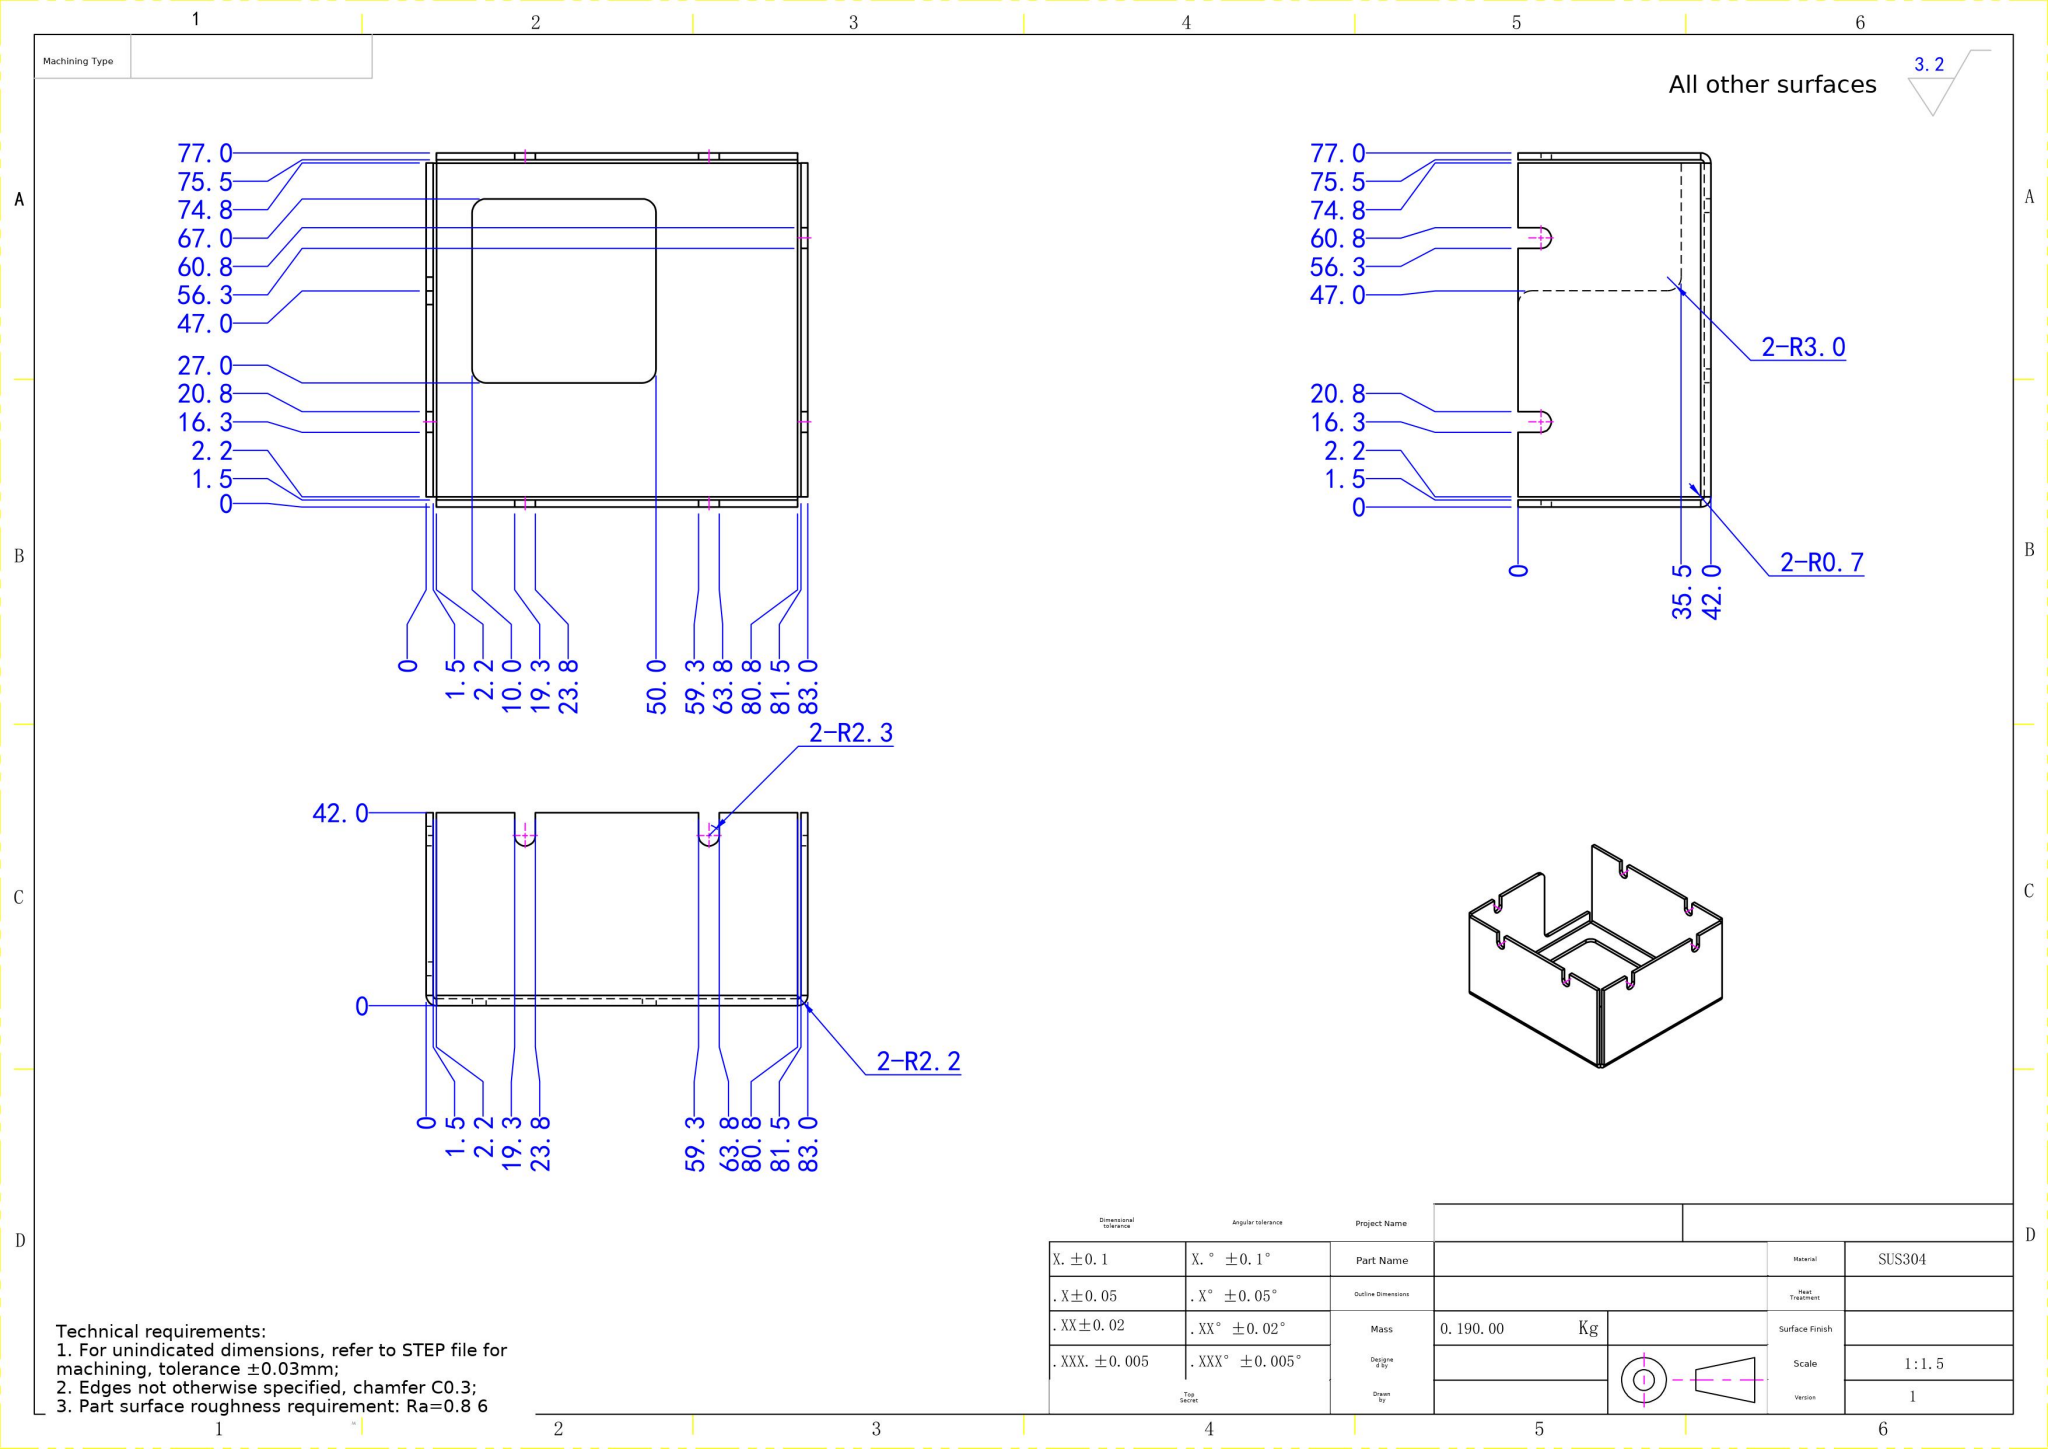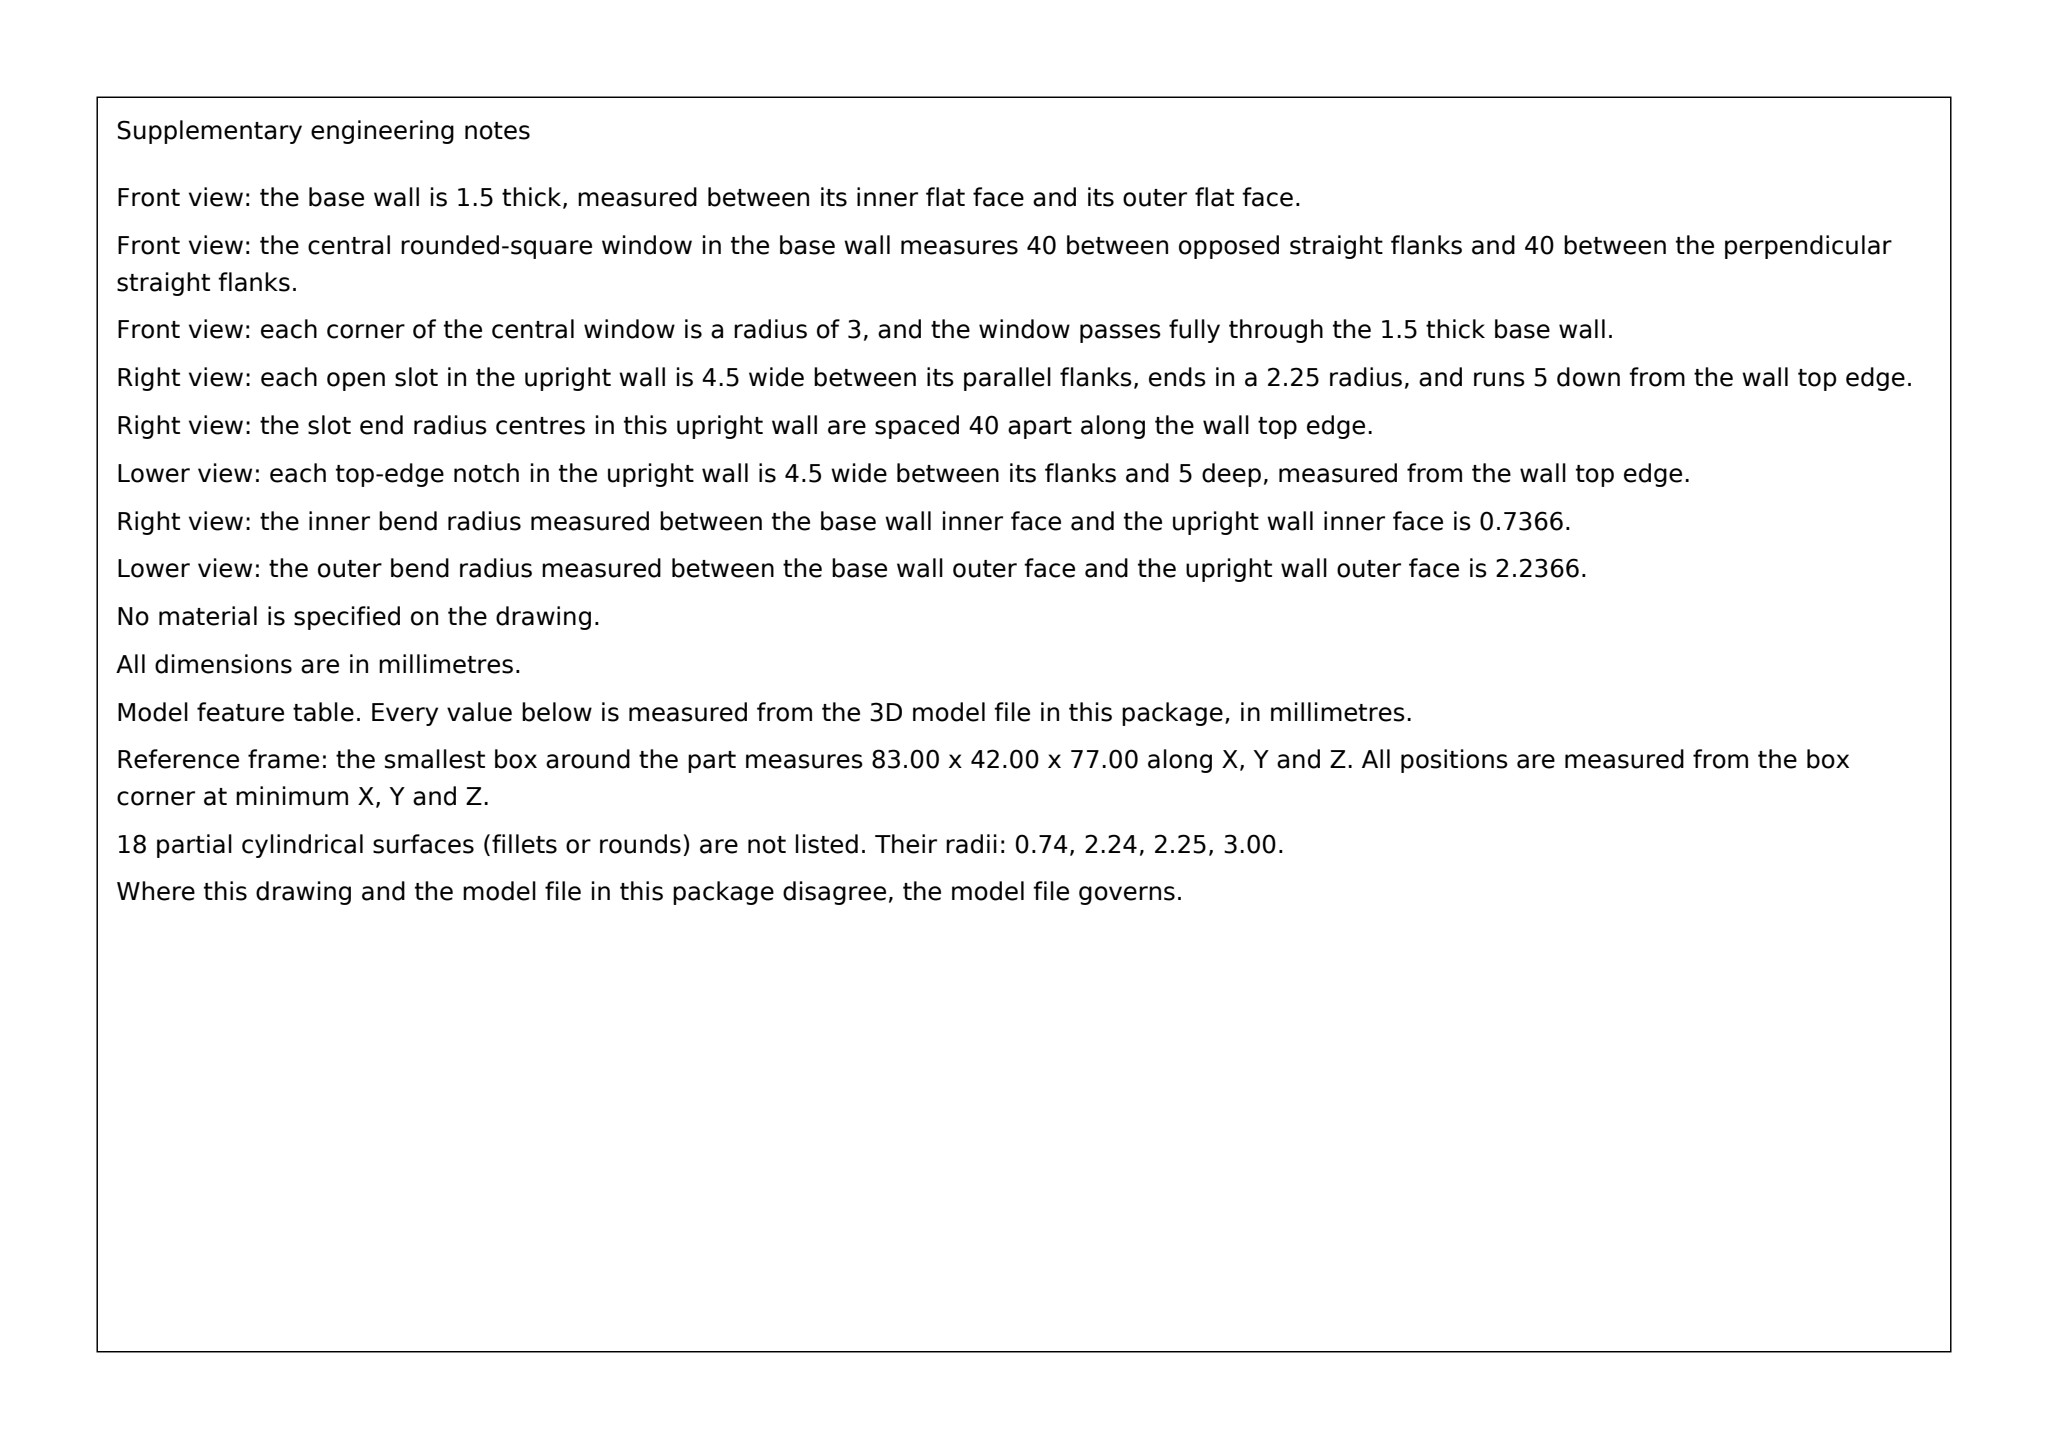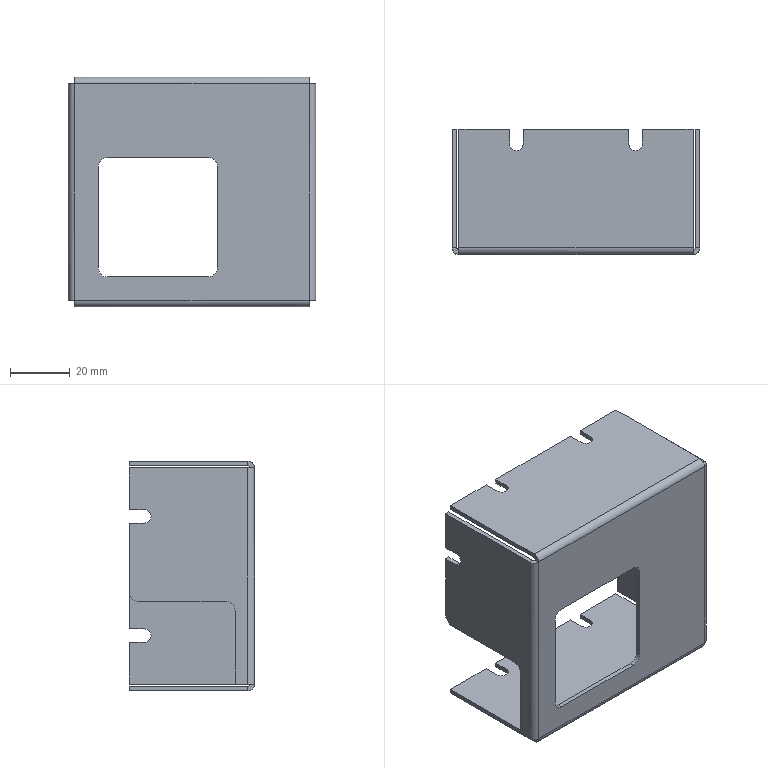Part | SolidWorks | mm | 1 solid | 81 faces | box 83 x 42 x 77 mm | volume 23447 mm3 | plane 49 | cylinder 24 | spline 8 | commonest cylinder face diameters 4.5 x10 6 x6 4.473 x4 1.473 x4
Drawing notes:
TOP SLOTS 4.5 WIDE x 5.0 DEEP FROM 42.0 EDGE; R2.25 END C/L 37.0 | from the solid: Ø4.5 cyls at y=37.02 (x=21.52/61.52 & z=18.52/58.52), top face y=42.015 -> 5.0 deep, R2.25 ends
40 x 40 WINDOW (X10.0-50.0, Z10.0-50.0): 4-R3.0 CORNERS | from the solid: Four Ø6.0 y-axis cyls at (13.02,13.02),(13.02,47.02),(47.02,13.02),(47.02,47.02); planes x/z=10.02 & 50.02